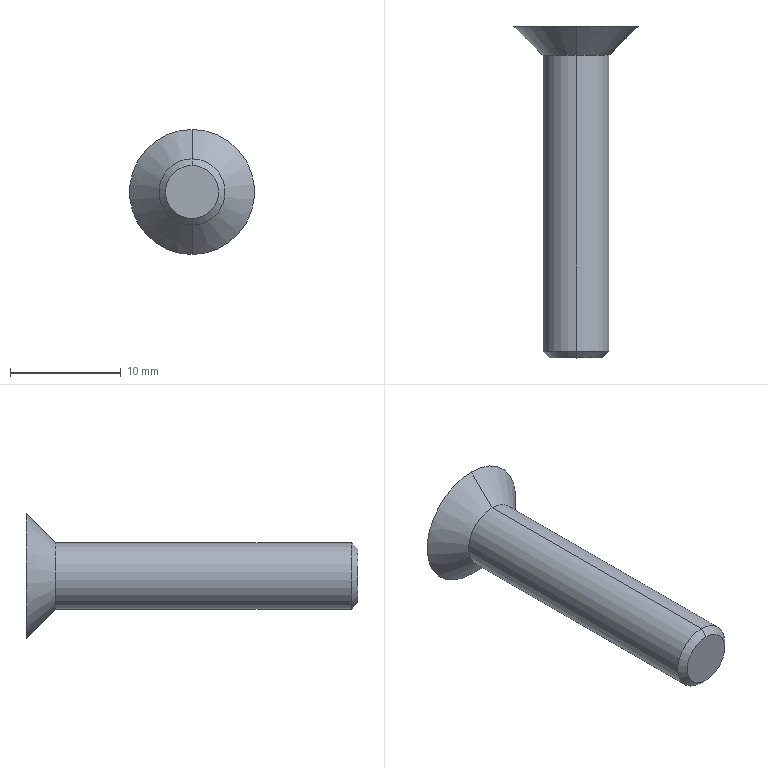Component | SolidWorks | SocketCountersunkHeadScrewM6x30-2 | 1 solid | 21 faces | box 11.3 x 30 x 11.3 mm | volume 911 mm3 | plane 15 | cone 4 | cylinder 2 | commonest cylinder face diameters 6 x2
build123d program:
from build123d import *
from OCP.BRepFilletAPI import BRepFilletAPI_MakeChamfer

# Parameters (mm, degrees)
SKETCH4_R           = 3
BOSS_EXTRUDE2_DEPTH = 30
CUT_EXTRUDE1_DEPTH  = 2.2
CHAMFER3_SIZE       = 1.153
CHAMFER3_SIZE2      = 1.997
CHAMFER4_SIZE       = 0.6


with BuildPart() as part:
    # Sketch2 → Revolve1 (revolve)
    with BuildSketch(Plane.XY, mode=Mode.PRIVATE) as revolve1_sk:
        Polygon((0, -3.72), (0, 0), (5.65, 0), (1.93, -3.72), align=None)
    revolve(revolve1_sk.sketch.rotate(Axis((0, -3.72, 0), (0, 1, 0)), 90), axis=Axis((0, -3.72, 0), (0, 1, 0)))

    # Sketch4 → Boss-Extrude2 (add)
    with BuildSketch(Plane.XZ):
        with Locations(Location((0, 0, 0), (0, 0, 90))):
            Circle(SKETCH4_R)
    extrude(amount=BOSS_EXTRUDE2_DEPTH)

    # Sketch3 → Cut-Extrude1 (cut)
    with BuildSketch(Plane(origin=(0, 0, 0), x_dir=(1, 0, 0), z_dir=(0, 1, 0))):
        Polygon((2, 1.155), (0, 2.309), (-2, 1.155), (-2, -1.155), (0, -2.309), (2, -1.155), align=None)
    extrude(amount=-CUT_EXTRUDE1_DEPTH, mode=Mode.SUBTRACT)

    # Chamfer3: one chamfer whose edges measure the first distance from different faces: ONE call of the kernel's chamfer builder (chamfer() names one face for all edges)
    chamfer3_edges_1 = [part.edges().sort_by_distance(p)[0] for p in [
        (2, -2.2, 0),
    ]]
    chamfer3_side_1 = [part.faces().sort_by_distance(p)[0] for p in [
        (2, -1.1, 0),
    ]]
    chamfer3_edges_2 = [part.edges().sort_by_distance(p)[0] for p in [
        (1, -2.2, 1.732),
    ]]
    chamfer3_side_2 = [part.faces().sort_by_distance(p)[0] for p in [
        (1, -1.1, 1.732),
    ]]
    chamfer3_edges_3 = [part.edges().sort_by_distance(p)[0] for p in [
        (-1, -2.2, 1.732),
    ]]
    chamfer3_side_3 = [part.faces().sort_by_distance(p)[0] for p in [
        (-1, -1.1, 1.732),
    ]]
    chamfer3_edges_4 = [part.edges().sort_by_distance(p)[0] for p in [
        (-2, -2.2, 0),
    ]]
    chamfer3_side_4 = [part.faces().sort_by_distance(p)[0] for p in [
        (-2, -1.1, 0),
    ]]
    chamfer3_edges_5 = [part.edges().sort_by_distance(p)[0] for p in [
        (-1, -2.2, -1.732),
    ]]
    chamfer3_side_5 = [part.faces().sort_by_distance(p)[0] for p in [
        (-1, -1.1, -1.732),
    ]]
    chamfer3_edges_6 = [part.edges().sort_by_distance(p)[0] for p in [
        (1, -2.2, -1.732),
    ]]
    chamfer3_side_6 = [part.faces().sort_by_distance(p)[0] for p in [
        (1, -1.1, -1.732),
    ]]
    chamfer3 = BRepFilletAPI_MakeChamfer(part.part.solid().wrapped)
    for e in chamfer3_edges_1:
        chamfer3.Add(CHAMFER3_SIZE, CHAMFER3_SIZE2, e.wrapped, chamfer3_side_1[0].wrapped)  # the first distance lies on this face
    for e in chamfer3_edges_2:
        chamfer3.Add(CHAMFER3_SIZE, CHAMFER3_SIZE2, e.wrapped, chamfer3_side_2[0].wrapped)  # the first distance lies on this face
    for e in chamfer3_edges_3:
        chamfer3.Add(CHAMFER3_SIZE, CHAMFER3_SIZE2, e.wrapped, chamfer3_side_3[0].wrapped)  # the first distance lies on this face
    for e in chamfer3_edges_4:
        chamfer3.Add(CHAMFER3_SIZE, CHAMFER3_SIZE2, e.wrapped, chamfer3_side_4[0].wrapped)  # the first distance lies on this face
    for e in chamfer3_edges_5:
        chamfer3.Add(CHAMFER3_SIZE, CHAMFER3_SIZE2, e.wrapped, chamfer3_side_5[0].wrapped)  # the first distance lies on this face
    for e in chamfer3_edges_6:
        chamfer3.Add(CHAMFER3_SIZE, CHAMFER3_SIZE2, e.wrapped, chamfer3_side_6[0].wrapped)  # the first distance lies on this face
    add(Compound.cast(chamfer3.Shape()), mode=Mode.REPLACE)

    # Chamfer4
    chamfer4_edges = [part.edges().sort_by_distance(p)[0] for p in [
        (0, -30, -3),
    ]]
    chamfer(chamfer4_edges, length=CHAMFER4_SIZE)


solid = part.part

# Placed as in the assembly
solid = solid.moved(Location((-71.946, -18, 23), (0, 0, 0)))
STEP:
#1=COLOUR_RGB('',0.7922,0.8196,0.9333);
#2=FILL_AREA_STYLE_COLOUR('',#1);
#3=FILL_AREA_STYLE('',(#2));
#4=SURFACE_STYLE_FILL_AREA(#3);
#5=SURFACE_SIDE_STYLE('',(#4));
#6=SURFACE_STYLE_USAGE(.BOTH.,#5);
#7=PRESENTATION_STYLE_ASSIGNMENT((#6));
#8=CARTESIAN_POINT('',(-2.833,-1.89,0.811));
#9=VERTEX_POINT('',#8);
#10=CARTESIAN_POINT('',(-2.833,-1.89,1.));
#11=VERTEX_POINT('',#10);
#12=CARTESIAN_POINT('',(-2.833,-1.89,0.9055));
#13=DIRECTION('',(0.,-1.,0.));
#14=DIRECTION('',(0.,0.,-1.));
#15=AXIS2_PLACEMENT_3D('',#12,#13,#14);
#16=CIRCLE('',#15,0.09449);
#17=EDGE_CURVE('',#9,#11,#16,.T.);
#18=ORIENTED_EDGE('',*,*,#17,.F.);
#19=CARTESIAN_POINT('',(-2.833,-1.866,0.7874));
#20=VERTEX_POINT('',#19);
#21=CARTESIAN_POINT('',(-2.833,-1.89,0.811));
#22=DIRECTION('',(0.,0.7071,-0.7071));
#23=VECTOR('',#22,39.37);
#24=LINE('',#21,#23);
#25=EDGE_CURVE('',#9,#20,#24,.T.);
#26=ORIENTED_EDGE('',*,*,#25,.T.);
#27=CARTESIAN_POINT('',(-2.833,-1.866,1.024));
#28=VERTEX_POINT('',#27);
#29=CARTESIAN_POINT('',(-2.833,-1.866,0.9055));
#30=DIRECTION('',(0.,1.,0.));
#31=DIRECTION('',(0.,0.,-1.));
#32=AXIS2_PLACEMENT_3D('',#29,#30,#31);
#33=CIRCLE('',#32,0.1181);
#34=EDGE_CURVE('',#28,#20,#33,.T.);
#35=ORIENTED_EDGE('',*,*,#34,.F.);
#36=CARTESIAN_POINT('',(-2.833,-1.89,1.));
#37=DIRECTION('',(0.,0.7071,0.7071));
#38=VECTOR('',#37,39.37);
#39=LINE('',#36,#38);
#40=EDGE_CURVE('',#11,#28,#39,.T.);
#41=ORIENTED_EDGE('',*,*,#40,.F.);
#42=EDGE_LOOP('',(#18,#26,#35,#41));
#43=FACE_OUTER_BOUND('',#42,.T.);
#44=CARTESIAN_POINT('',(-2.833,-1.89,0.9055));
#45=DIRECTION('',(0.,1.,0.));
#46=DIRECTION('',(0.,0.,1.));
#47=AXIS2_PLACEMENT_3D('',#44,#45,#46);
#48=CONICAL_SURFACE('',#47,0.09449,0.7854);
#49=ADVANCED_FACE('',(#43),#48,.T.);
#50=ORIENTED_EDGE('',*,*,#34,.T.);
#51=CARTESIAN_POINT('',(-2.833,-0.813,0.7874));
#52=VERTEX_POINT('',#51);
#53=CARTESIAN_POINT('',(-2.833,-1.89,0.7874));
#54=DIRECTION('',(0.,1.,0.));
#55=VECTOR('',#54,39.37);
#56=LINE('',#53,#55);
#57=EDGE_CURVE('',#20,#52,#56,.T.);
#58=ORIENTED_EDGE('',*,*,#57,.T.);
#59=CARTESIAN_POINT('',(-2.833,-0.813,1.024));
#60=VERTEX_POINT('',#59);
#61=CARTESIAN_POINT('',(-2.833,-0.813,0.9055));
#62=DIRECTION('',(0.,1.,0.));
#63=DIRECTION('',(0.,0.,1.));
#64=AXIS2_PLACEMENT_3D('',#61,#62,#63);
#65=CIRCLE('',#64,0.1181);
#66=EDGE_CURVE('',#60,#52,#65,.T.);
#67=ORIENTED_EDGE('',*,*,#66,.F.);
#68=CARTESIAN_POINT('',(-2.833,-1.89,1.024));
#69=DIRECTION('',(0.,1.,0.));
#70=VECTOR('',#69,39.37);
#71=LINE('',#68,#70);
#72=EDGE_CURVE('',#28,#60,#71,.T.);
#73=ORIENTED_EDGE('',*,*,#72,.F.);
#74=EDGE_LOOP('',(#50,#58,#67,#73));
#75=FACE_OUTER_BOUND('',#74,.T.);
#76=CARTESIAN_POINT('',(-2.833,-1.89,0.9055));
#77=DIRECTION('',(0.,1.,0.));
#78=DIRECTION('',(0.,0.,1.));
#79=AXIS2_PLACEMENT_3D('',#76,#77,#78);
#80=CYLINDRICAL_SURFACE('',#79,0.1181);
#81=ADVANCED_FACE('',(#75),#80,.T.);
#82=ORIENTED_EDGE('',*,*,#66,.T.);
#83=CARTESIAN_POINT('',(-2.833,-0.7087,0.6831));
#84=VERTEX_POINT('',#83);
#85=CARTESIAN_POINT('',(-2.833,-0.8551,0.8295));
#86=DIRECTION('',(0.,0.7071,-0.7071));
#87=VECTOR('',#86,39.37);
#88=LINE('',#85,#87);
#89=EDGE_CURVE('',#52,#84,#88,.T.);
#90=ORIENTED_EDGE('',*,*,#89,.T.);
#91=CARTESIAN_POINT('',(-2.833,-0.7087,1.128));
#92=VERTEX_POINT('',#91);
#93=CARTESIAN_POINT('',(-2.833,-0.7087,0.9055));
#94=DIRECTION('',(0.,-1.,0.));
#95=DIRECTION('',(0.,0.,-1.));
#96=AXIS2_PLACEMENT_3D('',#93,#94,#95);
#97=CIRCLE('',#96,0.2224);
#98=EDGE_CURVE('',#84,#92,#97,.T.);
#99=ORIENTED_EDGE('',*,*,#98,.T.);
#100=CARTESIAN_POINT('',(-2.833,-0.8551,0.9815));
#101=DIRECTION('',(0.,0.7071,0.7071));
#102=VECTOR('',#101,39.37);
#103=LINE('',#100,#102);
#104=EDGE_CURVE('',#60,#92,#103,.T.);
#105=ORIENTED_EDGE('',*,*,#104,.F.);
#106=EDGE_LOOP('',(#82,#90,#99,#105));
#107=FACE_OUTER_BOUND('',#106,.T.);
#108=CARTESIAN_POINT('',(-2.833,-0.8551,0.9055));
#109=DIRECTION('',(0.,1.,0.));
#110=DIRECTION('',(0.,0.,1.));
#111=AXIS2_PLACEMENT_3D('',#108,#109,#110);
#112=CONICAL_SURFACE('',#111,0.07598,0.7854);
#113=ADVANCED_FACE('',(#107),#112,.T.);
#114=ORIENTED_EDGE('',*,*,#89,.F.);
#115=CARTESIAN_POINT('',(-2.833,-0.813,0.9055));
#116=DIRECTION('',(0.,1.,0.));
#117=DIRECTION('',(0.,0.,1.));
#118=AXIS2_PLACEMENT_3D('',#115,#116,#117);
#119=CIRCLE('',#118,0.1181);
#120=EDGE_CURVE('',#52,#60,#119,.T.);
#121=ORIENTED_EDGE('',*,*,#120,.T.);
#122=ORIENTED_EDGE('',*,*,#104,.T.);
#123=CARTESIAN_POINT('',(-2.833,-0.7087,0.9055));
#124=DIRECTION('',(0.,-1.,0.));
#125=DIRECTION('',(0.,0.,-1.));
#126=AXIS2_PLACEMENT_3D('',#123,#124,#125);
#127=CIRCLE('',#126,0.2224);
#128=EDGE_CURVE('',#92,#84,#127,.T.);
#129=ORIENTED_EDGE('',*,*,#128,.T.);
#130=EDGE_LOOP('',(#114,#121,#122,#129));
#131=FACE_OUTER_BOUND('',#130,.T.);
#132=CARTESIAN_POINT('',(-2.833,-0.8551,0.9055));
#133=DIRECTION('',(0.,1.,0.));
#134=DIRECTION('',(0.,0.,1.));
#135=AXIS2_PLACEMENT_3D('',#132,#133,#134);
#136=CONICAL_SURFACE('',#135,0.07598,0.7854);
#137=ADVANCED_FACE('',(#131),#136,.T.);
#138=CARTESIAN_POINT('',(-2.754,-0.7087,0.951));
#139=VERTEX_POINT('',#138);
#140=CARTESIAN_POINT('',(-2.754,-0.7087,0.8601));
#141=VERTEX_POINT('',#140);
#142=CARTESIAN_POINT('',(-2.754,-0.7087,0.951));
#143=DIRECTION('',(-0.,0.,-1.));
#144=VECTOR('',#143,39.37);
#145=LINE('',#142,#144);
#146=EDGE_CURVE('',#139,#141,#145,.T.);
#147=ORIENTED_EDGE('',*,*,#146,.F.);
#148=CARTESIAN_POINT('',(-2.833,-0.7087,0.9964));
#149=VERTEX_POINT('',#148);
#150=CARTESIAN_POINT('',(-2.833,-0.7087,0.9964));
#151=DIRECTION('',(0.866,0.,-0.5));
#152=VECTOR('',#151,39.37);
#153=LINE('',#150,#152);
#154=EDGE_CURVE('',#149,#139,#153,.T.);
#155=ORIENTED_EDGE('',*,*,#154,.F.);
#156=CARTESIAN_POINT('',(-2.911,-0.7087,0.951));
#157=VERTEX_POINT('',#156);
#158=CARTESIAN_POINT('',(-2.911,-0.7087,0.951));
#159=DIRECTION('',(0.866,0.,0.5));
#160=VECTOR('',#159,39.37);
#161=LINE('',#158,#160);
#162=EDGE_CURVE('',#157,#149,#161,.T.);
#163=ORIENTED_EDGE('',*,*,#162,.F.);
#164=CARTESIAN_POINT('',(-2.911,-0.7087,0.8601));
#165=VERTEX_POINT('',#164);
#166=CARTESIAN_POINT('',(-2.911,-0.7087,0.8601));
#167=DIRECTION('',(0.,0.,1.));
#168=VECTOR('',#167,39.37);
#169=LINE('',#166,#168);
#170=EDGE_CURVE('',#165,#157,#169,.T.);
#171=ORIENTED_EDGE('',*,*,#170,.F.);
#172=CARTESIAN_POINT('',(-2.833,-0.7087,0.8146));
#173=VERTEX_POINT('',#172);
#174=CARTESIAN_POINT('',(-2.833,-0.7087,0.8146));
#175=DIRECTION('',(-0.866,0.,0.5));
#176=VECTOR('',#175,39.37);
#177=LINE('',#174,#176);
#178=EDGE_CURVE('',#173,#165,#177,.T.);
#179=ORIENTED_EDGE('',*,*,#178,.F.);
#180=CARTESIAN_POINT('',(-2.754,-0.7087,0.8601));
#181=DIRECTION('',(-0.866,0.,-0.5));
#182=VECTOR('',#181,39.37);
#183=LINE('',#180,#182);
#184=EDGE_CURVE('',#141,#173,#183,.T.);
#185=ORIENTED_EDGE('',*,*,#184,.F.);
#186=EDGE_LOOP('',(#147,#155,#163,#171,#179,#185));
#187=FACE_BOUND('',#186,.T.);
#188=ORIENTED_EDGE('',*,*,#128,.F.);
#189=ORIENTED_EDGE('',*,*,#98,.F.);
#190=EDGE_LOOP('',(#188,#189));
#191=FACE_OUTER_BOUND('',#190,.T.);
#192=CARTESIAN_POINT('',(-2.833,-0.7087,0.9055));
#193=DIRECTION('',(0.,1.,0.));
#194=DIRECTION('',(0.,0.,1.));
#195=AXIS2_PLACEMENT_3D('',#192,#193,#194);
#196=PLANE('',#195);
#197=ADVANCED_FACE('',(#187,#191),#196,.T.);
#198=ORIENTED_EDGE('',*,*,#57,.F.);
#199=CARTESIAN_POINT('',(-2.833,-1.866,0.9055));
#200=DIRECTION('',(0.,1.,0.));
#201=DIRECTION('',(0.,0.,-1.));
#202=AXIS2_PLACEMENT_3D('',#199,#200,#201);
#203=CIRCLE('',#202,0.1181);
#204=EDGE_CURVE('',#20,#28,#203,.T.);
#205=ORIENTED_EDGE('',*,*,#204,.T.);
#206=ORIENTED_EDGE('',*,*,#72,.T.);
#207=ORIENTED_EDGE('',*,*,#120,.F.);
#208=EDGE_LOOP('',(#198,#205,#206,#207));
#209=FACE_OUTER_BOUND('',#208,.T.);
#210=CARTESIAN_POINT('',(-2.833,-1.89,0.9055));
#211=DIRECTION('',(0.,1.,0.));
#212=DIRECTION('',(0.,0.,1.));
#213=AXIS2_PLACEMENT_3D('',#210,#211,#212);
#214=CYLINDRICAL_SURFACE('',#213,0.1181);
#215=ADVANCED_FACE('',(#209),#214,.T.);
#216=CARTESIAN_POINT('',(-2.833,-1.89,0.9055));
#217=DIRECTION('',(0.,-1.,0.));
#218=DIRECTION('',(0.,0.,-1.));
#219=AXIS2_PLACEMENT_3D('',#216,#217,#218);
#220=CIRCLE('',#219,0.09449);
#221=EDGE_CURVE('',#11,#9,#220,.T.);
#222=ORIENTED_EDGE('',*,*,#221,.T.);
#223=ORIENTED_EDGE('',*,*,#17,.T.);
#224=EDGE_LOOP('',(#222,#223));
#225=FACE_OUTER_BOUND('',#224,.T.);
#226=CARTESIAN_POINT('',(-2.833,-1.89,0.9055));
#227=DIRECTION('',(0.,-1.,0.));
#228=DIRECTION('',(0.,0.,-1.));
#229=AXIS2_PLACEMENT_3D('',#226,#227,#228);
#230=PLANE('',#229);
#231=ADVANCED_FACE('',(#225),#230,.T.);
#232=CARTESIAN_POINT('',(-2.754,-0.7499,0.8601));
#233=VERTEX_POINT('',#232);
#234=CARTESIAN_POINT('',(-2.754,-0.7953,0.8601));
#235=DIRECTION('',(0.,1.,0.));
#236=VECTOR('',#235,39.37);
#237=LINE('',#234,#236);
#238=EDGE_CURVE('',#233,#141,#237,.T.);
#239=ORIENTED_EDGE('',*,*,#238,.F.);
#240=CARTESIAN_POINT('',(-2.754,-0.7499,0.951));
#241=VERTEX_POINT('',#240);
#242=CARTESIAN_POINT('',(-2.754,-0.7499,0.951));
#243=DIRECTION('',(0.,0.,1.));
#244=VECTOR('',#243,39.37);
#245=LINE('',#242,#244);
#246=EDGE_CURVE('',#233,#241,#245,.T.);
#247=ORIENTED_EDGE('',*,*,#246,.T.);
#248=CARTESIAN_POINT('',(-2.754,-0.7953,0.951));
#249=DIRECTION('',(0.,1.,0.));
#250=VECTOR('',#249,39.37);
#251=LINE('',#248,#250);
#252=EDGE_CURVE('',#241,#139,#251,.T.);
#253=ORIENTED_EDGE('',*,*,#252,.T.);
#254=ORIENTED_EDGE('',*,*,#146,.T.);
#255=EDGE_LOOP('',(#239,#247,#253,#254));
#256=FACE_OUTER_BOUND('',#255,.T.);
#257=CARTESIAN_POINT('',(-2.754,-0.7953,0.951));
#258=DIRECTION('',(1.,0.,-0.));
#259=DIRECTION('',(-0.,0.,-1.));
#260=AXIS2_PLACEMENT_3D('',#257,#258,#259);
#261=PLANE('',#260);
#262=ADVANCED_FACE('',(#256),#261,.F.);
#263=ORIENTED_EDGE('',*,*,#252,.F.);
#264=CARTESIAN_POINT('',(-2.833,-0.7499,0.9964));
#265=VERTEX_POINT('',#264);
#266=CARTESIAN_POINT('',(-2.833,-0.7499,0.9964));
#267=DIRECTION('',(-0.866,0.,0.5));
#268=VECTOR('',#267,39.37);
#269=LINE('',#266,#268);
#270=EDGE_CURVE('',#241,#265,#269,.T.);
#271=ORIENTED_EDGE('',*,*,#270,.T.);
#272=CARTESIAN_POINT('',(-2.833,-0.7953,0.9964));
#273=DIRECTION('',(0.,1.,0.));
#274=VECTOR('',#273,39.37);
#275=LINE('',#272,#274);
#276=EDGE_CURVE('',#265,#149,#275,.T.);
#277=ORIENTED_EDGE('',*,*,#276,.T.);
#278=ORIENTED_EDGE('',*,*,#154,.T.);
#279=EDGE_LOOP('',(#263,#271,#277,#278));
#280=FACE_OUTER_BOUND('',#279,.T.);
#281=CARTESIAN_POINT('',(-2.833,-0.7953,0.9964));
#282=DIRECTION('',(0.5,0.,0.866));
#283=DIRECTION('',(0.866,0.,-0.5));
#284=AXIS2_PLACEMENT_3D('',#281,#282,#283);
#285=PLANE('',#284);
#286=ADVANCED_FACE('',(#280),#285,.F.);
#287=ORIENTED_EDGE('',*,*,#276,.F.);
#288=CARTESIAN_POINT('',(-2.911,-0.7499,0.951));
#289=VERTEX_POINT('',#288);
#290=CARTESIAN_POINT('',(-2.911,-0.7499,0.951));
#291=DIRECTION('',(-0.866,0.,-0.5));
#292=VECTOR('',#291,39.37);
#293=LINE('',#290,#292);
#294=EDGE_CURVE('',#265,#289,#293,.T.);
#295=ORIENTED_EDGE('',*,*,#294,.T.);
#296=CARTESIAN_POINT('',(-2.911,-0.7953,0.951));
#297=DIRECTION('',(0.,1.,0.));
#298=VECTOR('',#297,39.37);
#299=LINE('',#296,#298);
#300=EDGE_CURVE('',#289,#157,#299,.T.);
#301=ORIENTED_EDGE('',*,*,#300,.T.);
#302=ORIENTED_EDGE('',*,*,#162,.T.);
#303=EDGE_LOOP('',(#287,#295,#301,#302));
#304=FACE_OUTER_BOUND('',#303,.T.);
#305=CARTESIAN_POINT('',(-2.911,-0.7953,0.951));
#306=DIRECTION('',(-0.5,0.,0.866));
#307=DIRECTION('',(0.866,0.,0.5));
#308=AXIS2_PLACEMENT_3D('',#305,#306,#307);
#309=PLANE('',#308);
#310=ADVANCED_FACE('',(#304),#309,.F.);
#311=ORIENTED_EDGE('',*,*,#300,.F.);
#312=CARTESIAN_POINT('',(-2.911,-0.7499,0.8601));
#313=VERTEX_POINT('',#312);
#314=CARTESIAN_POINT('',(-2.911,-0.7499,0.8601));
#315=DIRECTION('',(0.,0.,-1.));
#316=VECTOR('',#315,39.37);
#317=LINE('',#314,#316);
#318=EDGE_CURVE('',#289,#313,#317,.T.);
#319=ORIENTED_EDGE('',*,*,#318,.T.);
#320=CARTESIAN_POINT('',(-2.911,-0.7953,0.8601));
#321=DIRECTION('',(0.,1.,0.));
#322=VECTOR('',#321,39.37);
#323=LINE('',#320,#322);
#324=EDGE_CURVE('',#313,#165,#323,.T.);
#325=ORIENTED_EDGE('',*,*,#324,.T.);
#326=ORIENTED_EDGE('',*,*,#170,.T.);
#327=EDGE_LOOP('',(#311,#319,#325,#326));
#328=FACE_OUTER_BOUND('',#327,.T.);
#329=CARTESIAN_POINT('',(-2.911,-0.7953,0.8601));
#330=DIRECTION('',(-1.,0.,0.));
#331=DIRECTION('',(0.,0.,1.));
#332=AXIS2_PLACEMENT_3D('',#329,#330,#331);
#333=PLANE('',#332);
#334=ADVANCED_FACE('',(#328),#333,.F.);
#335=ORIENTED_EDGE('',*,*,#324,.F.);
#336=CARTESIAN_POINT('',(-2.833,-0.7499,0.8146));
#337=VERTEX_POINT('',#336);
#338=CARTESIAN_POINT('',(-2.833,-0.7499,0.8146));
#339=DIRECTION('',(0.866,0.,-0.5));
#340=VECTOR('',#339,39.37);
#341=LINE('',#338,#340);
#342=EDGE_CURVE('',#313,#337,#341,.T.);
#343=ORIENTED_EDGE('',*,*,#342,.T.);
#344=CARTESIAN_POINT('',(-2.833,-0.7953,0.8146));
#345=DIRECTION('',(0.,1.,0.));
#346=VECTOR('',#345,39.37);
#347=LINE('',#344,#346);
#348=EDGE_CURVE('',#337,#173,#347,.T.);
#349=ORIENTED_EDGE('',*,*,#348,.T.);
#350=ORIENTED_EDGE('',*,*,#178,.T.);
#351=EDGE_LOOP('',(#335,#343,#349,#350));
#352=FACE_OUTER_BOUND('',#351,.T.);
#353=CARTESIAN_POINT('',(-2.833,-0.7953,0.8146));
#354=DIRECTION('',(-0.5,0.,-0.866));
#355=DIRECTION('',(-0.866,0.,0.5));
#356=AXIS2_PLACEMENT_3D('',#353,#354,#355);
#357=PLANE('',#356);
#358=ADVANCED_FACE('',(#352),#357,.F.);
#359=ORIENTED_EDGE('',*,*,#348,.F.);
#360=CARTESIAN_POINT('',(-2.754,-0.7499,0.8601));
#361=DIRECTION('',(0.866,0.,0.5));
#362=VECTOR('',#361,39.37);
#363=LINE('',#360,#362);
#364=EDGE_CURVE('',#337,#233,#363,.T.);
#365=ORIENTED_EDGE('',*,*,#364,.T.);
#366=ORIENTED_EDGE('',*,*,#238,.T.);
#367=ORIENTED_EDGE('',*,*,#184,.T.);
#368=EDGE_LOOP('',(#359,#365,#366,#367));
#369=FACE_OUTER_BOUND('',#368,.T.);
#370=CARTESIAN_POINT('',(-2.754,-0.7953,0.8601));
#371=DIRECTION('',(0.5,0.,-0.866));
#372=DIRECTION('',(-0.866,0.,-0.5));
#373=AXIS2_PLACEMENT_3D('',#370,#371,#372);
#374=PLANE('',#373);
#375=ADVANCED_FACE('',(#369),#374,.F.);
#376=CARTESIAN_POINT('',(-2.833,-0.7953,0.9054));
#377=VERTEX_POINT('',#376);
#378=CARTESIAN_POINT('',(-2.833,-0.7953,0.9056));
#379=VERTEX_POINT('',#378);
#380=CARTESIAN_POINT('',(-2.833,-0.7953,0.9055));
#381=DIRECTION('',(0.,0.,1.));
#382=VECTOR('',#381,39.37);
#383=LINE('',#380,#382);
#384=EDGE_CURVE('',#377,#379,#383,.T.);
#385=ORIENTED_EDGE('',*,*,#384,.T.);
#386=CARTESIAN_POINT('',(-2.833,-0.7953,0.9057));
#387=VERTEX_POINT('',#386);
#388=CARTESIAN_POINT('',(-2.833,-0.7953,0.9056));
#389=DIRECTION('',(0.866,0.,0.5));
#390=VECTOR('',#389,39.37);
#391=LINE('',#388,#390);
#392=EDGE_CURVE('',#379,#387,#391,.T.);
#393=ORIENTED_EDGE('',*,*,#392,.T.);
#394=CARTESIAN_POINT('',(-2.832,-0.7953,0.9056));
#395=VERTEX_POINT('',#394);
#396=CARTESIAN_POINT('',(-2.832,-0.7953,0.9056));
#397=DIRECTION('',(0.866,0.,-0.5));
#398=VECTOR('',#397,39.37);
#399=LINE('',#396,#398);
#400=EDGE_CURVE('',#387,#395,#399,.T.);
#401=ORIENTED_EDGE('',*,*,#400,.T.);
#402=CARTESIAN_POINT('',(-2.832,-0.7953,0.9054));
#403=VERTEX_POINT('',#402);
#404=CARTESIAN_POINT('',(-2.832,-0.7953,0.9055));
#405=DIRECTION('',(-0.,0.,-1.));
#406=VECTOR('',#405,39.37);
#407=LINE('',#404,#406);
#408=EDGE_CURVE('',#395,#403,#407,.T.);
#409=ORIENTED_EDGE('',*,*,#408,.T.);
#410=CARTESIAN_POINT('',(-2.833,-0.7953,0.9054));
#411=VERTEX_POINT('',#410);
#412=CARTESIAN_POINT('',(-2.832,-0.7953,0.9054));
#413=DIRECTION('',(-0.866,0.,-0.5));
#414=VECTOR('',#413,39.37);
#415=LINE('',#412,#414);
#416=EDGE_CURVE('',#403,#411,#415,.T.);
#417=ORIENTED_EDGE('',*,*,#416,.T.);
#418=CARTESIAN_POINT('',(-2.833,-0.7953,0.9054));
#419=DIRECTION('',(-0.866,0.,0.5));
#420=VECTOR('',#419,39.37);
#421=LINE('',#418,#420);
#422=EDGE_CURVE('',#411,#377,#421,.T.);
#423=ORIENTED_EDGE('',*,*,#422,.T.);
#424=EDGE_LOOP('',(#385,#393,#401,#409,#417,#423));
#425=FACE_OUTER_BOUND('',#424,.T.);
#426=CARTESIAN_POINT('',(-2.833,-0.7953,0.9055));
#427=DIRECTION('',(0.,1.,0.));
#428=DIRECTION('',(0.,0.,1.));
#429=AXIS2_PLACEMENT_3D('',#426,#427,#428);
#430=PLANE('',#429);
#431=ADVANCED_FACE('',(#425),#430,.T.);
#432=CARTESIAN_POINT('',(-2.832,-0.7953,0.9054));
#433=DIRECTION('',(-0.7746,-0.4472,0.4472));
#434=VECTOR('',#433,39.37);
#435=LINE('',#432,#434);
#436=EDGE_CURVE('',#233,#403,#435,.T.);
#437=ORIENTED_EDGE('',*,*,#436,.F.);
#438=ORIENTED_EDGE('',*,*,#364,.F.);
#439=CARTESIAN_POINT('',(-2.833,-0.7953,0.9054));
#440=DIRECTION('',(-0.,0.4472,-0.8944));
#441=VECTOR('',#440,39.37);
#442=LINE('',#439,#441);
#443=EDGE_CURVE('',#411,#337,#442,.T.);
#444=ORIENTED_EDGE('',*,*,#443,.F.);
#445=ORIENTED_EDGE('',*,*,#416,.F.);
#446=EDGE_LOOP('',(#437,#438,#444,#445));
#447=FACE_OUTER_BOUND('',#446,.T.);
#448=CARTESIAN_POINT('',(-2.832,-0.7953,0.9054));
#449=DIRECTION('',(0.25,-0.866,-0.433));
#450=DIRECTION('',(-0.866,0.,-0.5));
#451=AXIS2_PLACEMENT_3D('',#448,#449,#450);
#452=PLANE('',#451);
#453=ADVANCED_FACE('',(#447),#452,.F.);
#454=ORIENTED_EDGE('',*,*,#443,.T.);
#455=ORIENTED_EDGE('',*,*,#342,.F.);
#456=CARTESIAN_POINT('',(-2.833,-0.7953,0.9054));
#457=DIRECTION('',(-0.7746,0.4472,-0.4472));
#458=VECTOR('',#457,39.37);
#459=LINE('',#456,#458);
#460=EDGE_CURVE('',#377,#313,#459,.T.);
#461=ORIENTED_EDGE('',*,*,#460,.F.);
#462=ORIENTED_EDGE('',*,*,#422,.F.);
#463=EDGE_LOOP('',(#454,#455,#461,#462));
#464=FACE_OUTER_BOUND('',#463,.T.);
#465=CARTESIAN_POINT('',(-2.833,-0.7953,0.9054));
#466=DIRECTION('',(-0.25,-0.866,-0.433));
#467=DIRECTION('',(-0.866,0.,0.5));
#468=AXIS2_PLACEMENT_3D('',#465,#466,#467);
#469=PLANE('',#468);
#470=ADVANCED_FACE('',(#464),#469,.F.);
#471=ORIENTED_EDGE('',*,*,#436,.T.);
#472=ORIENTED_EDGE('',*,*,#408,.F.);
#473=CARTESIAN_POINT('',(-2.832,-0.7953,0.9056));
#474=DIRECTION('',(-0.7746,-0.4472,-0.4472));
#475=VECTOR('',#474,39.37);
#476=LINE('',#473,#475);
#477=EDGE_CURVE('',#241,#395,#476,.T.);
#478=ORIENTED_EDGE('',*,*,#477,.F.);
#479=ORIENTED_EDGE('',*,*,#246,.F.);
#480=EDGE_LOOP('',(#471,#472,#478,#479));
#481=FACE_OUTER_BOUND('',#480,.T.);
#482=CARTESIAN_POINT('',(-2.832,-0.7953,0.9055));
#483=DIRECTION('',(0.5,-0.866,-0.));
#484=DIRECTION('',(-0.,0.,-1.));
#485=AXIS2_PLACEMENT_3D('',#482,#483,#484);
#486=PLANE('',#485);
#487=ADVANCED_FACE('',(#481),#486,.F.);
#488=ORIENTED_EDGE('',*,*,#460,.T.);
#489=ORIENTED_EDGE('',*,*,#318,.F.);
#490=CARTESIAN_POINT('',(-2.833,-0.7953,0.9056));
#491=DIRECTION('',(-0.7746,0.4472,0.4472));
#492=VECTOR('',#491,39.37);
#493=LINE('',#490,#492);
#494=EDGE_CURVE('',#379,#289,#493,.T.);
#495=ORIENTED_EDGE('',*,*,#494,.F.);
#496=ORIENTED_EDGE('',*,*,#384,.F.);
#497=EDGE_LOOP('',(#488,#489,#495,#496));
#498=FACE_OUTER_BOUND('',#497,.T.);
#499=CARTESIAN_POINT('',(-2.833,-0.7953,0.9055));
#500=DIRECTION('',(-0.5,-0.866,0.));
#501=DIRECTION('',(0.,0.,1.));
#502=AXIS2_PLACEMENT_3D('',#499,#500,#501);
#503=PLANE('',#502);
#504=ADVANCED_FACE('',(#498),#503,.F.);
#505=ORIENTED_EDGE('',*,*,#477,.T.);
#506=ORIENTED_EDGE('',*,*,#400,.F.);
#507=CARTESIAN_POINT('',(-2.833,-0.7953,0.9056));
#508=DIRECTION('',(0.,-0.4472,-0.8944));
#509=VECTOR('',#508,39.37);
#510=LINE('',#507,#509);
#511=EDGE_CURVE('',#265,#387,#510,.T.);
#512=ORIENTED_EDGE('',*,*,#511,.F.);
#513=ORIENTED_EDGE('',*,*,#270,.F.);
#514=EDGE_LOOP('',(#505,#506,#512,#513));
#515=FACE_OUTER_BOUND('',#514,.T.);
#516=CARTESIAN_POINT('',(-2.832,-0.7953,0.9056));
#517=DIRECTION('',(0.25,-0.866,0.433));
#518=DIRECTION('',(0.866,0.,-0.5));
#519=AXIS2_PLACEMENT_3D('',#516,#517,#518);
#520=PLANE('',#519);
#521=ADVANCED_FACE('',(#515),#520,.F.);
#522=ORIENTED_EDGE('',*,*,#494,.T.);
#523=ORIENTED_EDGE('',*,*,#294,.F.);
#524=ORIENTED_EDGE('',*,*,#511,.T.);
#525=ORIENTED_EDGE('',*,*,#392,.F.);
#526=EDGE_LOOP('',(#522,#523,#524,#525));
#527=FACE_OUTER_BOUND('',#526,.T.);
#528=CARTESIAN_POINT('',(-2.833,-0.7953,0.9056));
#529=DIRECTION('',(-0.25,-0.866,0.433));
#530=DIRECTION('',(0.866,0.,0.5));
#531=AXIS2_PLACEMENT_3D('',#528,#529,#530);
#532=PLANE('',#531);
#533=ADVANCED_FACE('',(#527),#532,.F.);
#534=ORIENTED_EDGE('',*,*,#25,.F.);
#535=ORIENTED_EDGE('',*,*,#221,.F.);
#536=ORIENTED_EDGE('',*,*,#40,.T.);
#537=ORIENTED_EDGE('',*,*,#204,.F.);
#538=EDGE_LOOP('',(#534,#535,#536,#537));
#539=FACE_OUTER_BOUND('',#538,.T.);
#540=CARTESIAN_POINT('',(-2.833,-1.89,0.9055));
#541=DIRECTION('',(0.,1.,0.));
#542=DIRECTION('',(0.,0.,1.));
#543=AXIS2_PLACEMENT_3D('',#540,#541,#542);
#544=CONICAL_SURFACE('',#543,0.09449,0.7854);
#545=ADVANCED_FACE('',(#539),#544,.T.);
#546=CLOSED_SHELL('',(#49,#81,#113,#137,#197,#215,#231,#262,#286,#310,#334,#358,#375,#431,#453,#470,#487,#504,#521,#533,#545));
#547=MANIFOLD_SOLID_BREP('',#546);
#548=STYLED_ITEM('',(#7),#547);
#549=PRESENTATION_LAYER_ASSIGNMENT('','',(#548));
#550=CARTESIAN_POINT('',(0.,0.,0.));
#551=DIRECTION('',(0.,0.,1.));
#552=DIRECTION('',(1.,0.,0.));
#553=AXIS2_PLACEMENT_3D('',#550,#551,#552);
#554=(LENGTH_UNIT()NAMED_UNIT(*)SI_UNIT($,.METRE.));
#555=LENGTH_MEASURE_WITH_UNIT(LENGTH_MEASURE(0.0254),#554);
#556=DIMENSIONAL_EXPONENTS(1.,0.,0.,0.,0.,0.,0.);
#557=(CONVERSION_BASED_UNIT('',#555)LENGTH_UNIT()NAMED_UNIT(#556));
#558=UNCERTAINTY_MEASURE_WITH_UNIT(LENGTH_MEASURE(0.00001),#557,'','');
#559=(NAMED_UNIT(*)PLANE_ANGLE_UNIT()SI_UNIT($,.RADIAN.));
#560=(NAMED_UNIT(*)SI_UNIT($,.STERADIAN.)SOLID_ANGLE_UNIT());
#561=(GEOMETRIC_REPRESENTATION_CONTEXT(3)GLOBAL_UNCERTAINTY_ASSIGNED_CONTEXT((#558))GLOBAL_UNIT_ASSIGNED_CONTEXT((#557,#559,#560))REPRESENTATION_CONTEXT('',''));
#562=ADVANCED_BREP_SHAPE_REPRESENTATION('',(#547,#553),#561);
#563=(LENGTH_UNIT()NAMED_UNIT(*)SI_UNIT($,.METRE.));
#564=LENGTH_MEASURE_WITH_UNIT(LENGTH_MEASURE(0.0254),#563);
#565=DIMENSIONAL_EXPONENTS(1.,0.,0.,0.,0.,0.,0.);
#566=(CONVERSION_BASED_UNIT('',#564)LENGTH_UNIT()NAMED_UNIT(#565));
#567=UNCERTAINTY_MEASURE_WITH_UNIT(LENGTH_MEASURE(0.00001),#566,'','');
#568=(NAMED_UNIT(*)PLANE_ANGLE_UNIT()SI_UNIT($,.RADIAN.));
#569=(NAMED_UNIT(*)SI_UNIT($,.STERADIAN.)SOLID_ANGLE_UNIT());
#570=(GEOMETRIC_REPRESENTATION_CONTEXT(3)GLOBAL_UNCERTAINTY_ASSIGNED_CONTEXT((#567))GLOBAL_UNIT_ASSIGNED_CONTEXT((#566,#568,#569))REPRESENTATION_CONTEXT('',''));
#571=MECHANICAL_DESIGN_GEOMETRIC_PRESENTATION_REPRESENTATION('',(#548),#570);